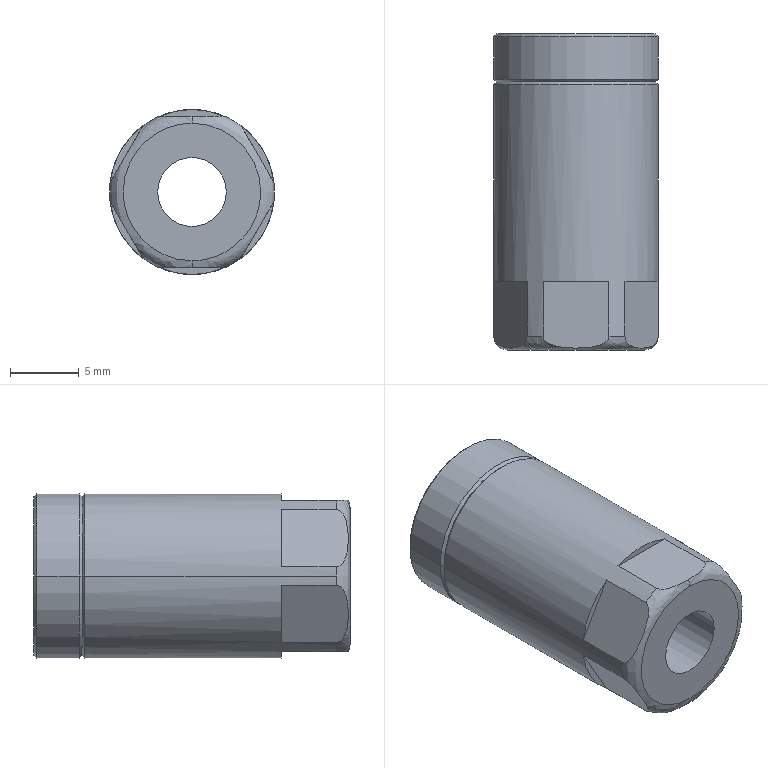Component | SolidWorks | MDJ16x20-10S_00_+-1_MDJ16x20-10S_00_+_4-1 | 1 solid | 31 faces | volume 1865 mm3 | plane 15 | cylinder 8 | cone 6 | spline 2 | commonest cylinder face diameters 12 x4 5 x2 6.5 x2